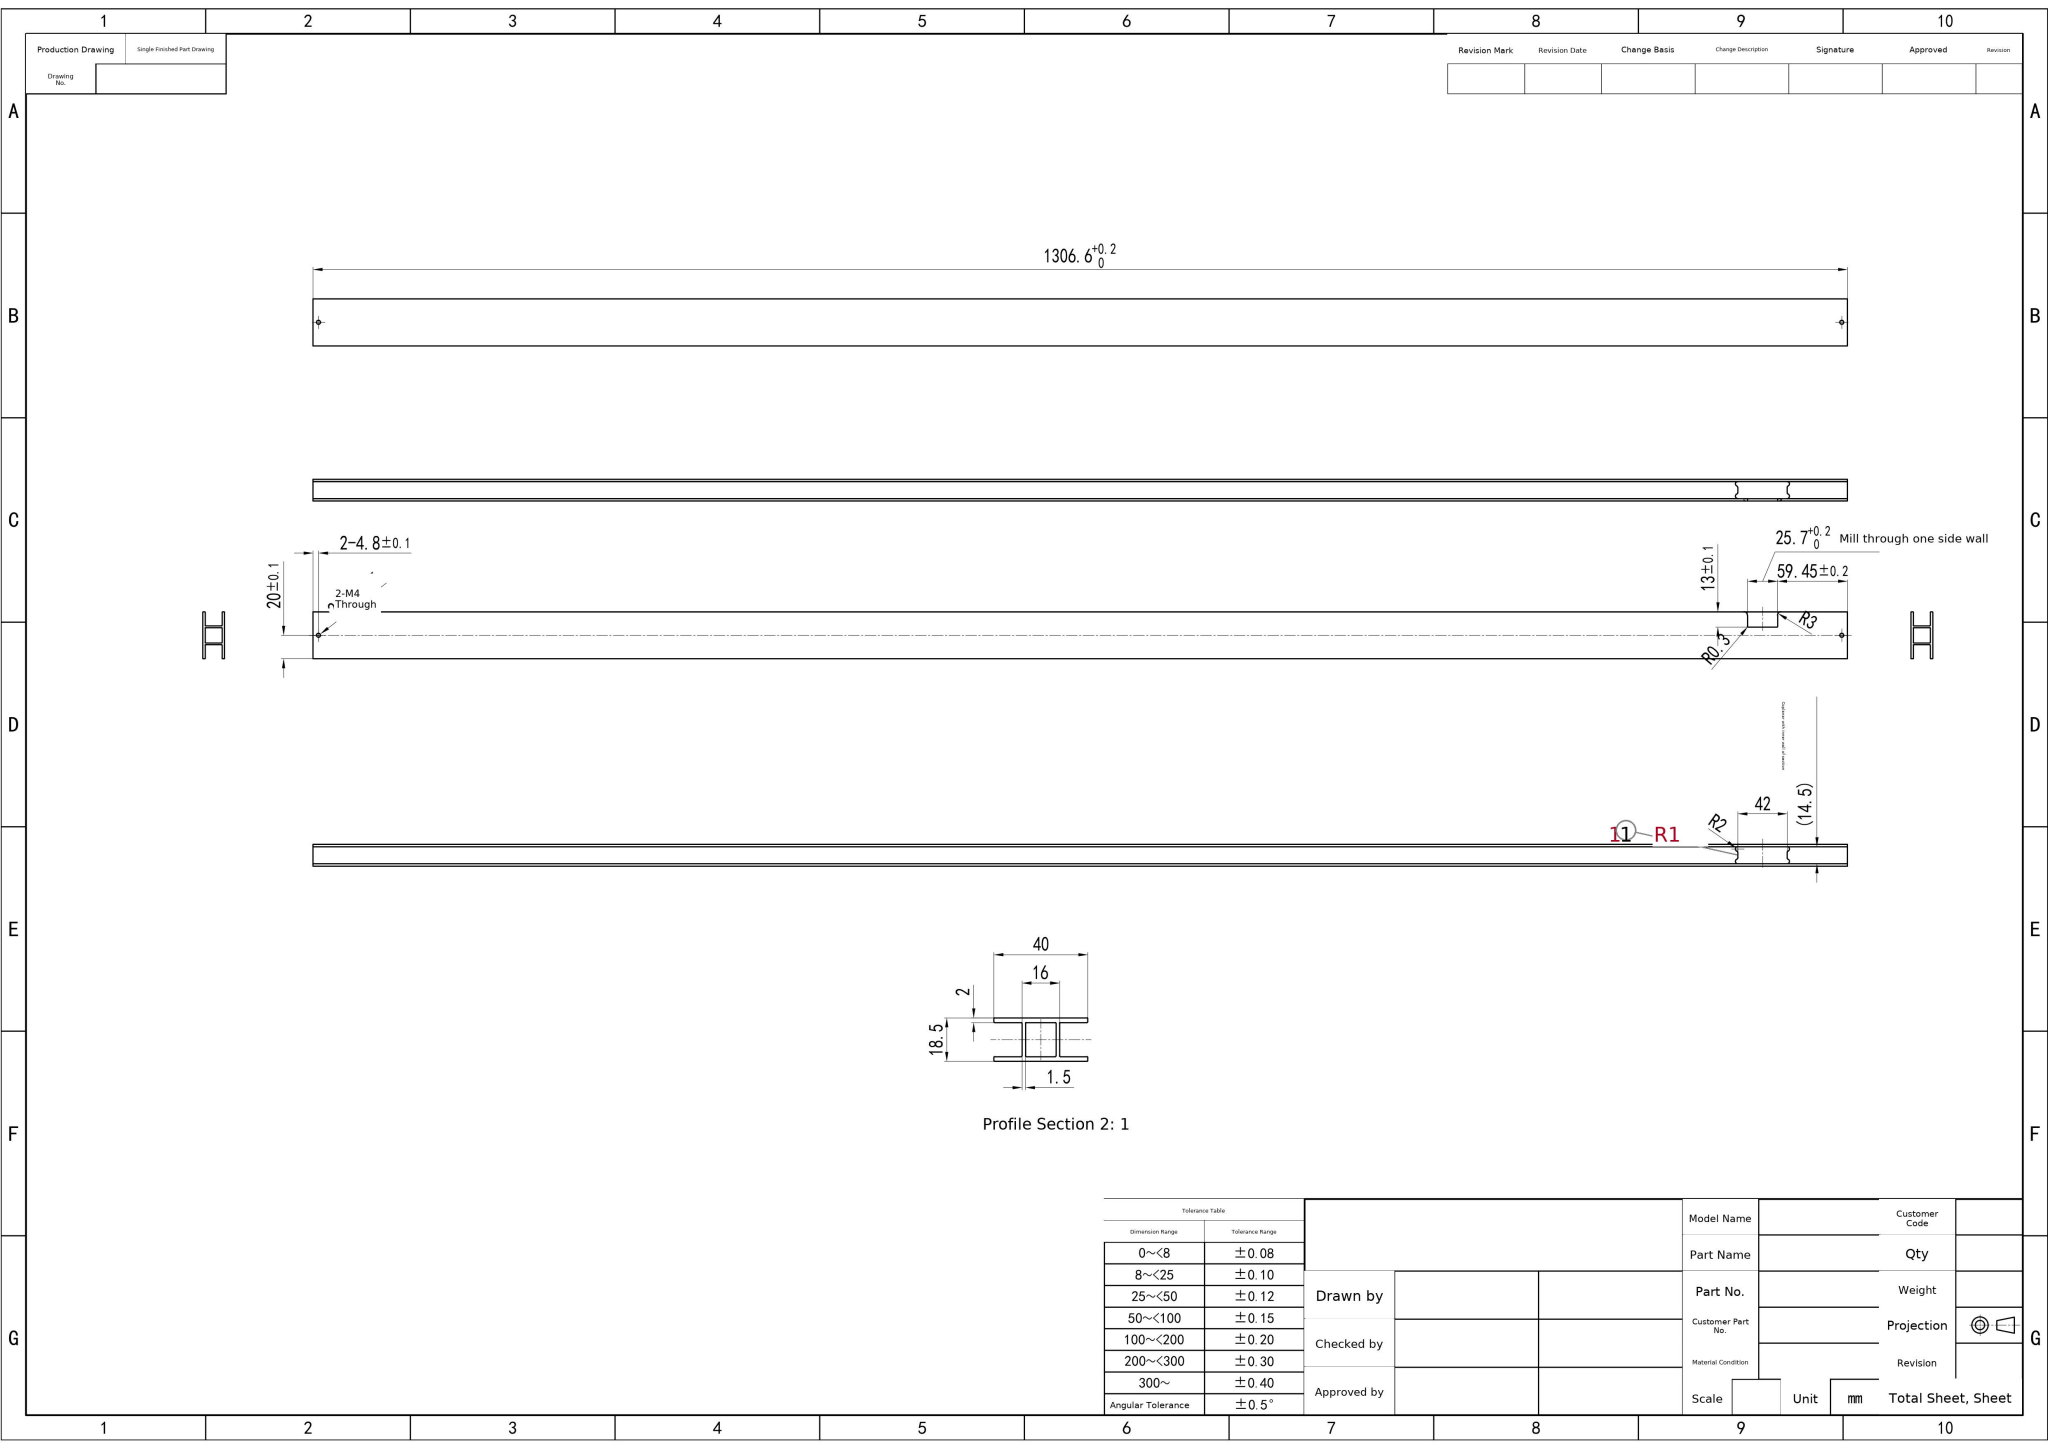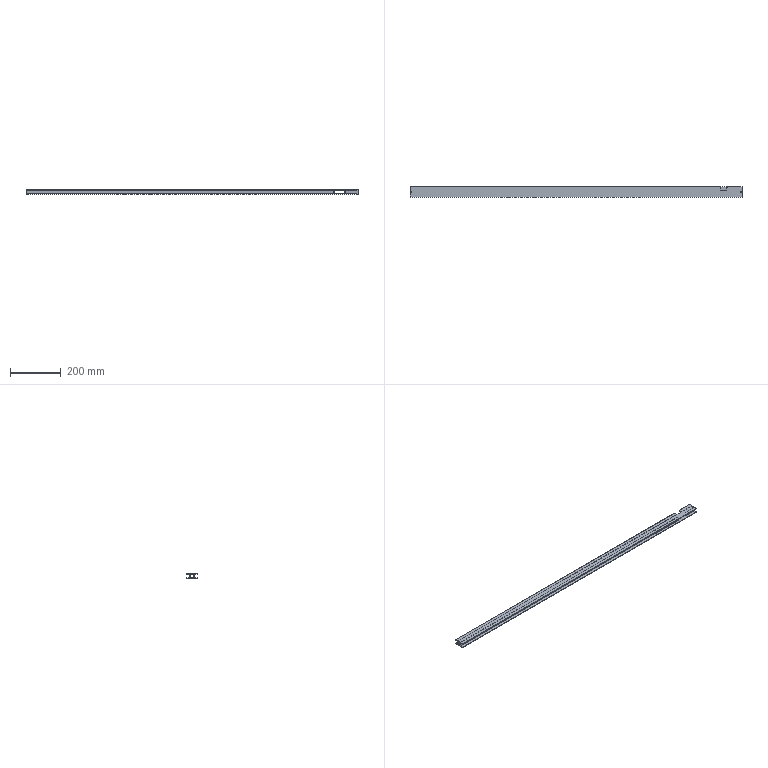Part | SolidWorks | mm | 1 solid | 80 faces | box 1306.6 x 40 x 18.5 mm | volume 263240 mm3 | cylinder 50 | plane 26 | spline 4 | commonest cylinder face diameters 0.6 x28 3.3 x8 4 x8 2 x4 6 x2